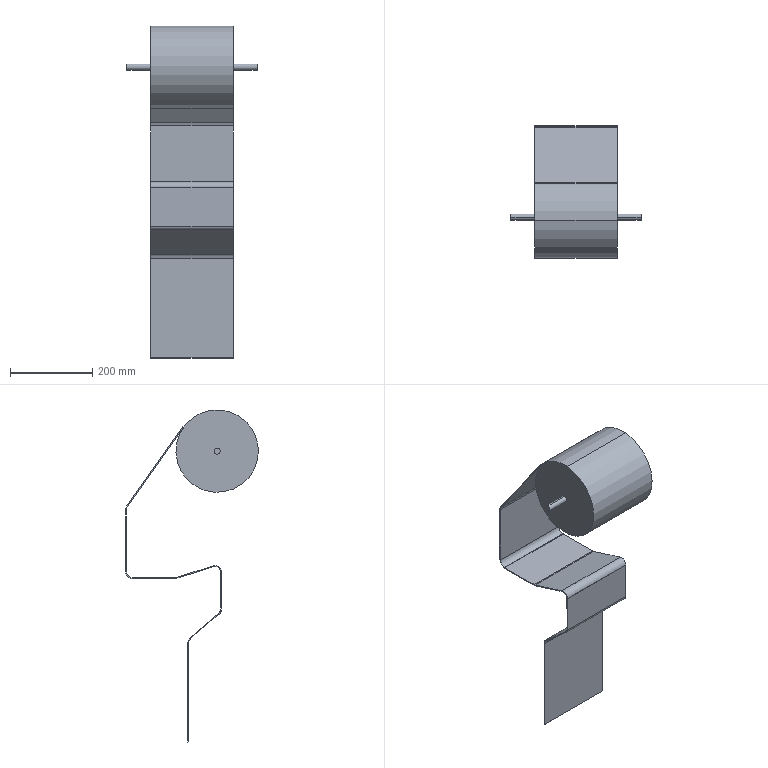Component | SolidWorks | Part6-1 | 2 solids | 42 faces | box 316 x 322.03 x 805.36 mm | volume 6741202 mm3 | plane 22 | cylinder 20 | commonest cylinder face diameters 30 x6 34 x5 15 x4 200 x2 20 x1 26 x1 16 x1
build123d program:
from build123d import *

# Parameters (mm, degrees)
SKETCH3_R           = 7.5
BOSS_EXTRUDE1_DEPTH = 158
SKETCH4_R           = 100
BOSS_EXTRUDE2_DEPTH = 100
EXTRUDE_THIN1_DEPTH = 100


with BuildPart() as part:
    # Sketch3 → Boss-Extrude1 (new, symmetric)
    with BuildSketch(Plane(origin=(0, 0, 0), x_dir=(0, 0, -1), z_dir=(1, 0, 0))):
        with Locations((107.861, 62.839)):
            Circle(SKETCH3_R)
    extrude(amount=BOSS_EXTRUDE1_DEPTH, both=True)

    # Sketch4 → Boss-Extrude2 (add, symmetric)
    with BuildSketch(Plane(origin=(0, 0, 0), x_dir=(0, 0, -1), z_dir=(1, 0, 0))):
        with Locations((107.861, 62.839)):
            Circle(SKETCH4_R)
    extrude(amount=BOSS_EXTRUDE2_DEPTH, both=True)

    # Sketch5 → Extrude-Thin1 (add, symmetric)
    with BuildSketch(Plane(origin=(0, 0, 0), x_dir=(0, 0, -1), z_dir=(1, 0, 0))):
        with BuildLine():
            Line((158.605, 149.008), (-43.77, 268.183))
            ThreePointArc((-43.77, 268.183), (-48.044, 269.882), (-52.632, 270.205))
            Line((-52.632, 270.205), (-202.109, 257.694))
            ThreePointArc((-202.109, 257.694), (-212.313, 252.431), (-215.806, 241.495))
            Line((-215.806, 241.495), (-207.465, 141.843))
            ThreePointArc((-207.465, 141.843), (-207.102, 139.589), (-206.401, 137.417))
            Line((-206.401, 137.417), (-170.292, 49.121))
            ThreePointArc((-170.292, 49.121), (-171.37, 35.632), (-182.869, 28.5))
            Line((-182.869, 28.5), (-275.238, 20.419))
            ThreePointArc((-275.238, 20.419), (-279.474, 20.963), (-283.097, 23.226))
            Line((-283.097, 23.226), (-349.764, 88.327))
            ThreePointArc((-349.764, 88.327), (-355.171, 91.711), (-361.495, 92.543))
            Line((-361.495, 92.543), (-533.642, 78.133))
            Line((-533.642, 78.133), (-600.775, 72.514))
            Line((-600.775, 72.514), (-600.942, 74.507))
            Line((-600.942, 74.507), (-533.809, 80.126))
            Line((-533.809, 80.126), (-361.662, 94.536))
            ThreePointArc((-361.662, 94.536), (-354.494, 93.593), (-348.367, 89.758))
            Line((-348.367, 89.758), (-281.699, 24.657))
            ThreePointArc((-281.699, 24.657), (-278.801, 22.847), (-275.413, 22.411))
            Line((-275.413, 22.411), (-183.043, 30.492))
            ThreePointArc((-183.043, 30.492), (-173.077, 36.674), (-172.143, 48.364))
            Line((-172.143, 48.364), (-208.252, 136.659))
            ThreePointArc((-208.252, 136.659), (-209.047, 139.122), (-209.458, 141.676))
            Line((-209.458, 141.676), (-217.799, 241.328))
            ThreePointArc((-217.799, 241.328), (-213.84, 253.722), (-202.276, 259.687))
            Line((-202.276, 259.687), (-52.799, 272.198))
            ThreePointArc((-52.799, 272.198), (-47.599, 271.832), (-42.755, 269.906))
            Line((-42.755, 269.906), (159.62, 150.732))
            Line((159.62, 150.732), (158.605, 149.008))
        make_face()
    extrude(amount=EXTRUDE_THIN1_DEPTH, both=True)


solid = part.part

# Placed as in the assembly
solid = solid.moved(Location((-6, 156.346, 214.514), (-175.215, 0, 180)))